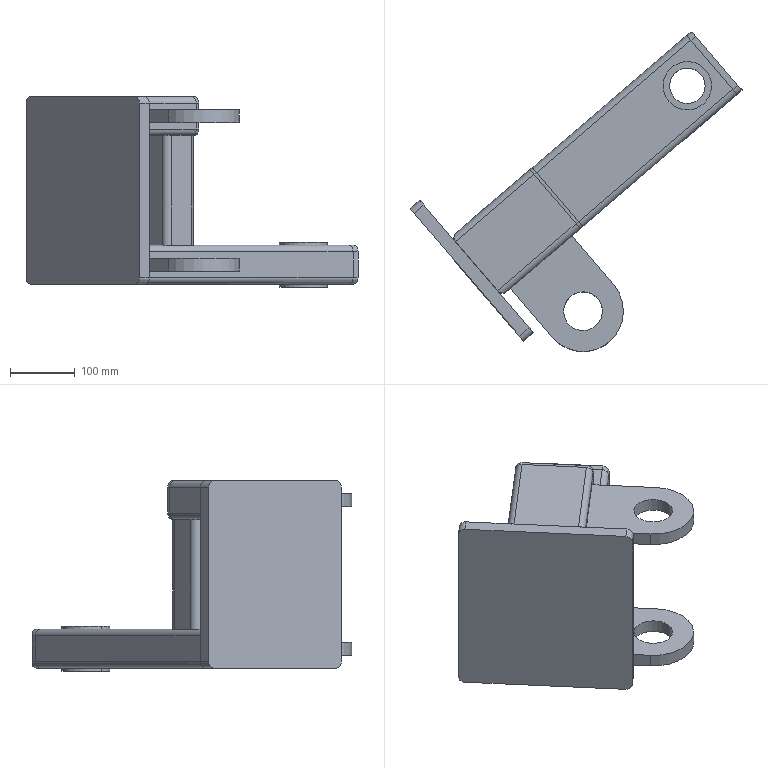Component | SolidWorks | CuttingMachineFrame-1 | 10 solids | 129 faces | box 514.07 x 494.46 x 295 mm | volume 4004790 mm3 | plane 71 | cylinder 58 | commonest cylinder face diameters 20 x28 10 x16 75 x6 60 x4 125 x2 55 x2 | material Stainless Steel
build123d program:
from build123d import *

# Parameters (mm, degrees)
RECTANGULAR_TUBE_CONFIGURED_70_X_40_X_DEPTH = 518.082
RECTANGULAR_TUBE_CONFIGURED_70_X_4_3_DEPTH  = 366.164
RECTANGULAR_TUBE_CONFIGURED_70_X_4_5_DEPTH  = 518.082
RECTANGULAR_TUBE_CONFIGURED_70_X_4_6_DEPTH  = 170
SKETCH4_R                                   = 37.5
CUT_EXTRUDE1_2_DEPTH                        = 565.004
BOSS_EXTRUDE1_DEPTH                         = 10
BOSS_EXTRUDE1_DEPTH_BACK                    = 10
SKETCH5_R                                   = 30
SKETCH6_R                                   = 37.5
SKETCH6_R_2                                 = 27.5
BOSS_EXTRUDE2_DEPTH                         = 70
SKETCH7_W                                   = 270
SKETCH7_H                                   = 290
BOSS_EXTRUDE3_DEPTH                         = 20
FILLET1_R                                   = 10
BOSS_EXTRUDE4_DEPTH                         = 10
BOSS_EXTRUDE4_2_DEPTH                       = 10
SKETCH9_W                                   = 330
SKETCH9_H                                   = 70
CUT_EXTRUDE2_DEPTH                          = 633.48
BOSS_EXTRUDE6_DEPTH                         = 5
CUT_EXTRUDE1_DEPTH                          = 609.055
CUT_EXTRUDE1_DEPTH_BACK                     = 609.055


with BuildPart() as part:
    # Sketch1 → Rectangular tube - configured 70 X 40 X (new body)
    with BuildSketch(Plane.YZ):
        with BuildLine():
            Line((-20, -60), (20, -60))
            ThreePointArc((20, -60), (27.071, -57.071), (30, -50))
            Line((30, -50), (30, 50))
            ThreePointArc((30, 50), (27.071, 57.071), (20, 60))
            Line((20, 60), (-20, 60))
            ThreePointArc((-20, 60), (-27.071, 57.071), (-30, 50))
            Line((-30, 50), (-30, -50))
            ThreePointArc((-30, -50), (-27.071, -57.071), (-20, -60))
        make_face()
        with BuildLine():
            Line((-20, -55), (20, -55))
            ThreePointArc((20, -55), (23.536, -53.536), (25, -50))
            Line((25, -50), (25, 50))
            ThreePointArc((25, 50), (23.536, 53.536), (20, 55))
            Line((20, 55), (-20, 55))
            ThreePointArc((-20, 55), (-23.536, 53.536), (-25, 50))
            Line((-25, 50), (-25, -50))
            ThreePointArc((-25, -50), (-23.536, -53.536), (-20, -55))
        make_face(mode=Mode.SUBTRACT)
    extrude(amount=RECTANGULAR_TUBE_CONFIGURED_70_X_40_X_DEPTH)

    # Rectangular tube - configured 70 X 4 2
    split(bisect_by=Plane(origin=(450, 0, 0), x_dir=(-0.7071, -0.7071, 0), z_dir=(-0.7071, 0.7071, 0)), keep=Keep.TOP)


with BuildPart() as body_2:
    # Sketch1 on segment 2 (on carried to segment 2) → Rectangular tube - configured 70 X 4 3 (new body)
    with BuildSketch(Plane(origin=(450, 68.082, 0), x_dir=(1, 0, 0), z_dir=(0, -1, 0))):
        with BuildLine():
            Line((-20, -60), (20, -60))
            ThreePointArc((20, -60), (27.071, -57.071), (30, -50))
            Line((30, -50), (30, 50))
            ThreePointArc((30, 50), (27.071, 57.071), (20, 60))
            Line((20, 60), (-20, 60))
            ThreePointArc((-20, 60), (-27.071, 57.071), (-30, 50))
            Line((-30, 50), (-30, -50))
            ThreePointArc((-30, -50), (-27.071, -57.071), (-20, -60))
        make_face()
        with BuildLine():
            Line((-20, -55), (20, -55))
            ThreePointArc((20, -55), (23.536, -53.536), (25, -50))
            Line((25, -50), (25, 50))
            ThreePointArc((25, 50), (23.536, 53.536), (20, 55))
            Line((20, 55), (-20, 55))
            ThreePointArc((-20, 55), (-23.536, 53.536), (-25, 50))
            Line((-25, 50), (-25, -50))
            ThreePointArc((-25, -50), (-23.536, -53.536), (-20, -55))
        make_face(mode=Mode.SUBTRACT)
    extrude(amount=RECTANGULAR_TUBE_CONFIGURED_70_X_4_3_DEPTH)

    # Rectangular tube - configured 70 X 4 3 m
    split(bisect_by=Plane(origin=(450, 0, 0), x_dir=(0.7071, 0.7071, 0), z_dir=(0.7071, -0.7071, 0)), keep=Keep.TOP)

    # Rectangular tube - configured 70 X 4 4
    split(bisect_by=Plane(origin=(450, -230, 0), x_dir=(-0.7071, 0.7071, 0), z_dir=(0.7071, 0.7071, 0)), keep=Keep.TOP)


with BuildPart() as body_3:
    # Sketch1 on segment 3 (on carried to segment 3) → Rectangular tube - configured 70 X 4 5 (new body)
    with BuildSketch(Plane(origin=(518.082, -230, 0), x_dir=(0, -1, 0), z_dir=(-1, 0, 0))):
        with BuildLine():
            Line((-20, -60), (20, -60))
            ThreePointArc((20, -60), (27.071, -57.071), (30, -50))
            Line((30, -50), (30, 50))
            ThreePointArc((30, 50), (27.071, 57.071), (20, 60))
            Line((20, 60), (-20, 60))
            ThreePointArc((-20, 60), (-27.071, 57.071), (-30, 50))
            Line((-30, 50), (-30, -50))
            ThreePointArc((-30, -50), (-27.071, -57.071), (-20, -60))
        make_face()
        with BuildLine():
            Line((-20, -55), (20, -55))
            ThreePointArc((20, -55), (23.536, -53.536), (25, -50))
            Line((25, -50), (25, 50))
            ThreePointArc((25, 50), (23.536, 53.536), (20, 55))
            Line((20, 55), (-20, 55))
            ThreePointArc((-20, 55), (-23.536, 53.536), (-25, 50))
            Line((-25, 50), (-25, -50))
            ThreePointArc((-25, -50), (-23.536, -53.536), (-20, -55))
        make_face(mode=Mode.SUBTRACT)
    extrude(amount=RECTANGULAR_TUBE_CONFIGURED_70_X_4_5_DEPTH)

    # Rectangular tube - configured 70 X 4 5 m
    split(bisect_by=Plane(origin=(450, -230, 0), x_dir=(0.7071, -0.7071, 0), z_dir=(-0.7071, -0.7071, 0)), keep=Keep.TOP)


with BuildPart() as body_4:
    # Sketch11 → Rectangular tube - configured 70 X 4 6 (new body)
    with BuildSketch(Plane(origin=(350, -30, 0), x_dir=(1, 0, 0), z_dir=(0, -1, 0))):
        with BuildLine():
            Line((-20, -60), (20, -60))
            ThreePointArc((20, -60), (27.071, -57.071), (30, -50))
            Line((30, -50), (30, 50))
            ThreePointArc((30, 50), (27.071, 57.071), (20, 60))
            Line((20, 60), (-20, 60))
            ThreePointArc((-20, 60), (-27.071, 57.071), (-30, 50))
            Line((-30, 50), (-30, -50))
            ThreePointArc((-30, -50), (-27.071, -57.071), (-20, -60))
        make_face()
        with BuildLine():
            Line((-20, -55), (20, -55))
            ThreePointArc((20, -55), (23.536, -53.536), (25, -50))
            Line((25, -50), (25, 50))
            ThreePointArc((25, 50), (23.536, 53.536), (20, 55))
            Line((20, 55), (-20, 55))
            ThreePointArc((-20, 55), (-23.536, 53.536), (-25, 50))
            Line((-25, 50), (-25, -50))
            ThreePointArc((-25, -50), (-23.536, -53.536), (-20, -55))
        make_face(mode=Mode.SUBTRACT)
    extrude(amount=RECTANGULAR_TUBE_CONFIGURED_70_X_4_6_DEPTH)


with BuildPart() as cut_extrude1_2_tool:
    # Sketch4 → Cut-Extrude1_2 (new, through all)
    with BuildSketch(Plane.XZ.offset(260)):
        with Locations((50, 0)):
            Circle(SKETCH4_R)
    extrude(amount=-CUT_EXTRUDE1_2_DEPTH)


with BuildPart() as part_1:
    add(part.part)

    # Cut-Extrude1_2: cut by cut_extrude1_2_tool
    add(cut_extrude1_2_tool.part, mode=Mode.SUBTRACT)


with BuildPart() as body_3_1:
    add(body_3.part)

    # Cut-Extrude1_2: cut by cut_extrude1_2_tool
    add(cut_extrude1_2_tool.part, mode=Mode.SUBTRACT)


with BuildPart() as body_5:
    # Sketch5 → Boss-Extrude1 (new, two sides: drawn at the far end of the back side and taken through both)
    with BuildSketch(Plane(origin=(0, 0, 0), x_dir=(1, 0, 0), z_dir=(0, 1, 0)).offset(-BOSS_EXTRUDE1_DEPTH_BACK)):
        with BuildLine():
            Line((462.5, 160), (462.5, 60))
            Line((462.5, 60), (337.5, 60))
            Line((337.5, 60), (337.5, 160))
            ThreePointArc((337.5, 160), (400, 222.5), (462.5, 160))
        make_face()
        with Locations(Location((400, 160, 0), (0, 0, 270))):
            Circle(SKETCH5_R, mode=Mode.SUBTRACT)
    extrude(amount=BOSS_EXTRUDE1_DEPTH + BOSS_EXTRUDE1_DEPTH_BACK)


with BuildPart() as body_6:
    # Mirror1: mirrored copy
    add(body_5.part.mirror(Plane.ZX.offset(-115)))


with BuildPart() as body_7:
    # Sketch6 → Boss-Extrude2 (new body)
    with BuildSketch(Plane(origin=(0, -265, 0), x_dir=(-1, 0, 0), z_dir=(0, -1, 0))):
        with Locations(Location((-50, 0, 0), (0, 0, 180))):
            Circle(SKETCH6_R)
        with Locations(Location((-50, 0, 0), (0, 0, 180))):
            Circle(SKETCH6_R_2, mode=Mode.SUBTRACT)
    extrude(amount=-BOSS_EXTRUDE2_DEPTH)


with BuildPart() as body_8:
    # Mirror2: mirrored copy
    add(body_7.part.mirror(Plane.ZX.offset(-115)))


with BuildPart() as body_9:
    # Sketch7 → Boss-Extrude3 (new body)
    with BuildSketch(Plane(origin=(480, 0, 0), x_dir=(0, 0, -1), z_dir=(1, 0, 0))):
        with Locations((0, -115)):
            Rectangle(SKETCH7_W, SKETCH7_H)
    extrude(amount=BOSS_EXTRUDE3_DEPTH)

    # Fillet1
    fillet1_edges = [body_9.edges().sort_by_distance(p)[0] for p in [
        (490, 30, 135),
        (490, 30, -135),
        (490, -260, -135),
        (490, -260, 135),
    ]]
    fillet(fillet1_edges, radius=FILLET1_R)


with BuildPart() as body_10:
    # Sketch8 → Boss-Extrude4 (new body)
    with BuildSketch(Plane.ZY):
        with BuildLine():
            Line((60, -250), (60, -210))
            ThreePointArc((60, -210), (57.071, -202.929), (50, -200))
            Line((50, -200), (-50, -200))
            ThreePointArc((-50, -200), (-57.071, -202.929), (-60, -210))
            Line((-60, -210), (-60, -250))
            ThreePointArc((-60, -250), (-57.071, -257.071), (-50, -260))
            Line((-50, -260), (50, -260))
            ThreePointArc((50, -260), (57.071, -257.071), (60, -250))
        make_face()
    extrude(amount=BOSS_EXTRUDE4_DEPTH)

    # Sketch12 → Cut-Extrude1 (cut, two sides: drawn at the far end of the back side and taken through both)
    with BuildSketch(Plane(origin=(0, 0, 0), x_dir=(1, 0, 0), z_dir=(0, 1, 0)).offset(-CUT_EXTRUDE1_DEPTH_BACK)):
        Polygon((-7, -60), (-10, -57), (-12, -62), align=None)
    extrude(amount=CUT_EXTRUDE1_DEPTH + CUT_EXTRUDE1_DEPTH_BACK, mode=Mode.SUBTRACT)


with BuildPart() as body_11:
    # Sketch8 → Boss-Extrude4 2 (new body)
    with BuildSketch(Plane.ZY):
        with BuildLine():
            Line((50, 30), (-50, 30))
            ThreePointArc((-50, 30), (-57.071, 27.071), (-60, 20))
            Line((-60, 20), (-60, -20))
            ThreePointArc((-60, -20), (-57.071, -27.071), (-50, -30))
            Line((-50, -30), (50, -30))
            ThreePointArc((50, -30), (57.071, -27.071), (60, -20))
            Line((60, -20), (60, 20))
            ThreePointArc((60, 20), (57.071, 27.071), (50, 30))
        make_face()
    extrude(amount=BOSS_EXTRUDE4_2_DEPTH)


with BuildPart() as cut_extrude2_tool:
    # Sketch9 → Cut-Extrude2 (new, through all)
    with BuildSketch(Plane.XY.offset(60)):
        with Locations((155, 0)):
            Rectangle(SKETCH9_W, SKETCH9_H)
    extrude(amount=-CUT_EXTRUDE2_DEPTH)


with BuildPart() as part_2:
    add(part_1.part)

    # Cut-Extrude2: cut by cut_extrude2_tool
    add(cut_extrude2_tool.part, mode=Mode.SUBTRACT)


with BuildPart() as body_8_1:
    add(body_8.part)

    # Cut-Extrude2: cut by cut_extrude2_tool
    add(cut_extrude2_tool.part, mode=Mode.SUBTRACT)


with BuildPart() as body_11_1:
    add(body_11.part)

    # Cut-Extrude2: cut by cut_extrude2_tool
    add(cut_extrude2_tool.part, mode=Mode.SUBTRACT)


with BuildPart() as body_10_2:
    # Sketch10 → Boss-Extrude6 (new body)
    with BuildSketch(Plane.ZY.offset(-320)):
        with BuildLine():
            Line((50, 30), (-50, 30))
            ThreePointArc((-50, 30), (-57.071, 27.071), (-60, 20))
            Line((-60, 20), (-60, -20))
            ThreePointArc((-60, -20), (-57.071, -27.071), (-50, -30))
            Line((-50, -30), (50, -30))
            ThreePointArc((50, -30), (57.071, -27.071), (60, -20))
            Line((60, -20), (60, 20))
            ThreePointArc((60, 20), (57.071, 27.071), (50, 30))
        make_face()
    extrude(amount=BOSS_EXTRUDE6_DEPTH)


solid = Compound([body_2.part, body_4.part, body_3_1.part, body_5.part, body_6.part, body_7.part, body_9.part, body_10.part, part_2.part, body_10_2.part])

# Placed as in the assembly
solid = solid.moved(Location((-335.213, 1349.312, 365.7), (-90, -40.619, -180)))